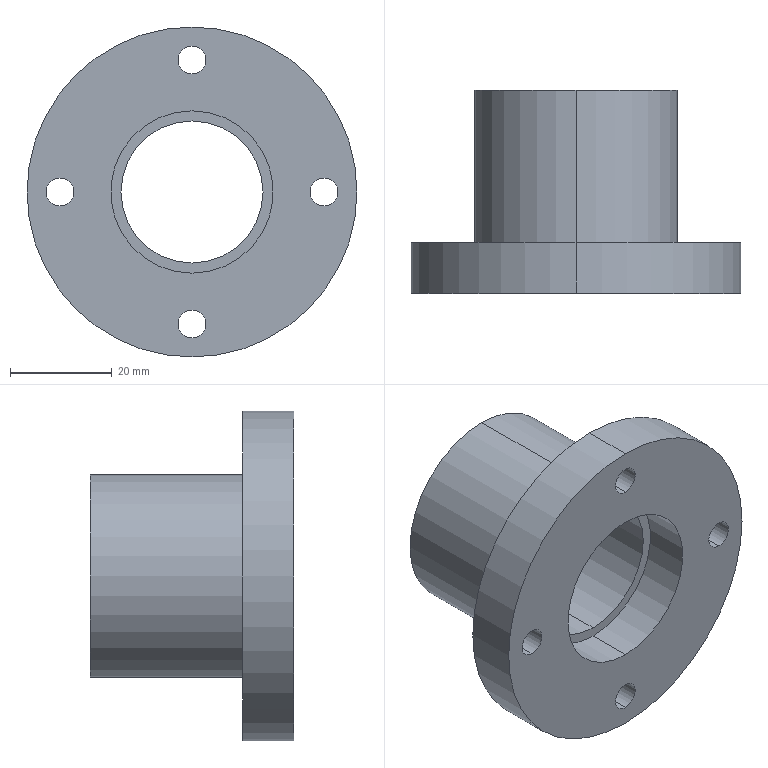Component | SolidWorks | 75-02-23StirringBearingHousing-1 | 1 solid | 35 faces | box 65 x 40 x 65 mm | volume 40660 mm3 | cylinder 26 | plane 9 | commonest cylinder face diameters 10 x8 5.5 x8 32 x4 40 x2 65 x2 28 x2 | material A3 Steel
build123d program:
from build123d import *

# Parameters (mm, degrees)
SKETCH1_R                                          = 32.5
BOSS_EXTRUDE1_DEPTH                                = 10
HOLE_SIZE_ACCORDING_TO_TYPE_OF_HEXAGON_D           = 5.5
HOLE_SIZE_ACCORDING_TO_TYPE_OF_HEXAGON_CBORE_D     = 10
HOLE_SIZE_ACCORDING_TO_TYPE_OF_HEXAGON_CBORE_DEPTH = 5.7
CIRPATTERN1_COUNT                                  = 4
SKETCH5_R                                          = 20
BOSS_EXTRUDE2_DEPTH                                = 30
SKETCH6_R                                          = 14
CUT_EXTRUDE1_DEPTH                                 = 61.93
SKETCH7_R                                          = 16
CUT_EXTRUDE2_DEPTH                                 = 9
CUT_EXTRUDE3_START                                 = -9
SKETCH8_R                                          = 16
CUT_EXTRUDE3_DEPTH                                 = 9


with BuildPart() as part:
    # Sketch1 → Boss-Extrude1 (new body)
    with BuildSketch(Plane.XY):
        Circle(SKETCH1_R)
    extrude(amount=BOSS_EXTRUDE1_DEPTH)

    # Hole Size _according to_ Type of Hexagon (through all)
    with Locations(Plane(origin=(26, 0, 0), x_dir=(-1, 0, 0), z_dir=(0, 0, -1))):
        with Locations((0, 0)):
            hole_size_according_to_type_of_hexagon = CounterBoreHole(HOLE_SIZE_ACCORDING_TO_TYPE_OF_HEXAGON_D / 2, HOLE_SIZE_ACCORDING_TO_TYPE_OF_HEXAGON_CBORE_D / 2, HOLE_SIZE_ACCORDING_TO_TYPE_OF_HEXAGON_CBORE_DEPTH)

    # CirPattern1: Hole Size _according to_ Type of Hexagon ×4 about axis
    cirpattern1_axis = Axis((0, 0, 0), (0, 0, 1))
    for i in range(1, CIRPATTERN1_COUNT):
        add(hole_size_according_to_type_of_hexagon.rotate(cirpattern1_axis, i * 360 / CIRPATTERN1_COUNT), mode=Mode.SUBTRACT)

    # Sketch5 → Boss-Extrude2 (add)
    with BuildSketch(Plane(origin=(0, 0, 0), x_dir=(-1, 0, 0), z_dir=(0, 0, -1))):
        with Locations(Location((0, 0, 0), (0, 0, 180))):
            Circle(SKETCH5_R)
    extrude(amount=BOSS_EXTRUDE2_DEPTH)

    # Sketch6 → Cut-Extrude1 (cut, through all)
    with BuildSketch(Plane(origin=(0, 0, -30), x_dir=(-1, 0, 0), z_dir=(0, 0, -1))):
        Circle(SKETCH6_R)
    extrude(amount=-CUT_EXTRUDE1_DEPTH, mode=Mode.SUBTRACT)

    # Sketch7 → Cut-Extrude2 (cut)
    with BuildSketch(Plane(origin=(0, 0, -30), x_dir=(-1, 0, 0), z_dir=(0, 0, -1))):
        Circle(SKETCH7_R)
    extrude(amount=-CUT_EXTRUDE2_DEPTH, mode=Mode.SUBTRACT)

    # Sketch8 → Cut-Extrude3 (cut)
    with BuildSketch(Plane.XY.offset(10).offset(CUT_EXTRUDE3_START)):
        with Locations(Location((0, 0, 0), (0, 0, 180))):
            Circle(SKETCH8_R)
    extrude(amount=CUT_EXTRUDE3_DEPTH, mode=Mode.SUBTRACT)


solid = part.part

# Placed as in the assembly
solid = solid.moved(Location((-17.87, 205.857, -43.68), (90, 0, 0)))
STEP:
#1=CARTESIAN_POINT('',(-0.7036,8.065,-2.35));
#2=VERTEX_POINT('',#1);
#3=CARTESIAN_POINT('',(-0.7036,8.065,-1.09));
#4=VERTEX_POINT('',#3);
#5=CARTESIAN_POINT('',(-0.7036,8.065,-1.72));
#6=DIRECTION('',(-0.,-1.,0.));
#7=DIRECTION('',(0.,0.,1.));
#8=AXIS2_PLACEMENT_3D('',#5,#6,#7);
#9=CIRCLE('',#8,0.6299);
#10=EDGE_CURVE('',#2,#4,#9,.T.);
#11=ORIENTED_EDGE('',*,*,#10,.F.);
#12=CARTESIAN_POINT('',(-0.7036,7.711,-2.35));
#13=VERTEX_POINT('',#12);
#14=CARTESIAN_POINT('',(-0.7036,8.065,-2.35));
#15=DIRECTION('',(-0.,-1.,0.));
#16=VECTOR('',#15,39.37);
#17=LINE('',#14,#16);
#18=EDGE_CURVE('',#2,#13,#17,.T.);
#19=ORIENTED_EDGE('',*,*,#18,.T.);
#20=CARTESIAN_POINT('',(-0.7036,7.711,-1.09));
#21=VERTEX_POINT('',#20);
#22=CARTESIAN_POINT('',(-0.7036,7.711,-1.72));
#23=DIRECTION('',(-0.,-1.,0.));
#24=DIRECTION('',(0.,0.,1.));
#25=AXIS2_PLACEMENT_3D('',#22,#23,#24);
#26=CIRCLE('',#25,0.6299);
#27=EDGE_CURVE('',#13,#21,#26,.T.);
#28=ORIENTED_EDGE('',*,*,#27,.T.);
#29=CARTESIAN_POINT('',(-0.7036,8.065,-1.09));
#30=DIRECTION('',(-0.,-1.,0.));
#31=VECTOR('',#30,39.37);
#32=LINE('',#29,#31);
#33=EDGE_CURVE('',#4,#21,#32,.T.);
#34=ORIENTED_EDGE('',*,*,#33,.F.);
#35=EDGE_LOOP('',(#11,#19,#28,#34));
#36=FACE_OUTER_BOUND('',#35,.T.);
#37=CARTESIAN_POINT('',(-0.7036,8.065,-1.72));
#38=DIRECTION('',(-0.,-1.,0.));
#39=DIRECTION('',(0.,0.,1.));
#40=AXIS2_PLACEMENT_3D('',#37,#38,#39);
#41=CYLINDRICAL_SURFACE('',#40,0.6299);
#42=ADVANCED_FACE('',(#36),#41,.F.);
#43=CARTESIAN_POINT('',(-0.7036,8.931,-1.09));
#44=VERTEX_POINT('',#43);
#45=CARTESIAN_POINT('',(-0.7036,8.931,-2.35));
#46=VERTEX_POINT('',#45);
#47=CARTESIAN_POINT('',(-0.7036,8.931,-1.72));
#48=DIRECTION('',(0.,1.,-0.));
#49=DIRECTION('',(-0.,0.,-1.));
#50=AXIS2_PLACEMENT_3D('',#47,#48,#49);
#51=CIRCLE('',#50,0.6299);
#52=EDGE_CURVE('',#44,#46,#51,.T.);
#53=ORIENTED_EDGE('',*,*,#52,.F.);
#54=CARTESIAN_POINT('',(-0.7036,9.286,-1.09));
#55=VERTEX_POINT('',#54);
#56=CARTESIAN_POINT('',(-0.7036,8.931,-1.09));
#57=DIRECTION('',(0.,1.,-0.));
#58=VECTOR('',#57,39.37);
#59=LINE('',#56,#58);
#60=EDGE_CURVE('',#44,#55,#59,.T.);
#61=ORIENTED_EDGE('',*,*,#60,.T.);
#62=CARTESIAN_POINT('',(-0.7036,9.286,-2.35));
#63=VERTEX_POINT('',#62);
#64=CARTESIAN_POINT('',(-0.7036,9.286,-1.72));
#65=DIRECTION('',(0.,1.,-0.));
#66=DIRECTION('',(-0.,0.,-1.));
#67=AXIS2_PLACEMENT_3D('',#64,#65,#66);
#68=CIRCLE('',#67,0.6299);
#69=EDGE_CURVE('',#55,#63,#68,.T.);
#70=ORIENTED_EDGE('',*,*,#69,.T.);
#71=CARTESIAN_POINT('',(-0.7036,8.931,-2.35));
#72=DIRECTION('',(0.,1.,-0.));
#73=VECTOR('',#72,39.37);
#74=LINE('',#71,#73);
#75=EDGE_CURVE('',#46,#63,#74,.T.);
#76=ORIENTED_EDGE('',*,*,#75,.F.);
#77=EDGE_LOOP('',(#53,#61,#70,#76));
#78=FACE_OUTER_BOUND('',#77,.T.);
#79=CARTESIAN_POINT('',(-0.7036,8.931,-1.72));
#80=DIRECTION('',(0.,1.,-0.));
#81=DIRECTION('',(-0.,0.,-1.));
#82=AXIS2_PLACEMENT_3D('',#79,#80,#81);
#83=CYLINDRICAL_SURFACE('',#82,0.6299);
#84=ADVANCED_FACE('',(#78),#83,.F.);
#85=CARTESIAN_POINT('',(-0.7036,9.286,-2.507));
#86=VERTEX_POINT('',#85);
#87=CARTESIAN_POINT('',(-0.7036,9.286,-0.9323));
#88=VERTEX_POINT('',#87);
#89=CARTESIAN_POINT('',(-0.7036,9.286,-1.72));
#90=DIRECTION('',(0.,1.,-0.));
#91=DIRECTION('',(-0.,0.,-1.));
#92=AXIS2_PLACEMENT_3D('',#89,#90,#91);
#93=CIRCLE('',#92,0.7874);
#94=EDGE_CURVE('',#86,#88,#93,.T.);
#95=ORIENTED_EDGE('',*,*,#94,.F.);
#96=CARTESIAN_POINT('',(-0.7036,8.105,-2.507));
#97=VERTEX_POINT('',#96);
#98=CARTESIAN_POINT('',(-0.7036,9.286,-2.507));
#99=DIRECTION('',(-0.,-1.,0.));
#100=VECTOR('',#99,39.37);
#101=LINE('',#98,#100);
#102=EDGE_CURVE('',#86,#97,#101,.T.);
#103=ORIENTED_EDGE('',*,*,#102,.T.);
#104=CARTESIAN_POINT('',(-0.7036,8.105,-0.9323));
#105=VERTEX_POINT('',#104);
#106=CARTESIAN_POINT('',(-0.7036,8.105,-1.72));
#107=DIRECTION('',(0.,1.,-0.));
#108=DIRECTION('',(0.,0.,1.));
#109=AXIS2_PLACEMENT_3D('',#106,#107,#108);
#110=CIRCLE('',#109,0.7874);
#111=EDGE_CURVE('',#97,#105,#110,.T.);
#112=ORIENTED_EDGE('',*,*,#111,.T.);
#113=CARTESIAN_POINT('',(-0.7036,9.286,-0.9323));
#114=DIRECTION('',(-0.,-1.,0.));
#115=VECTOR('',#114,39.37);
#116=LINE('',#113,#115);
#117=EDGE_CURVE('',#88,#105,#116,.T.);
#118=ORIENTED_EDGE('',*,*,#117,.F.);
#119=EDGE_LOOP('',(#95,#103,#112,#118));
#120=FACE_OUTER_BOUND('',#119,.T.);
#121=CARTESIAN_POINT('',(-0.7036,9.286,-1.72));
#122=DIRECTION('',(-0.,-1.,0.));
#123=DIRECTION('',(0.,0.,1.));
#124=AXIS2_PLACEMENT_3D('',#121,#122,#123);
#125=CYLINDRICAL_SURFACE('',#124,0.7874);
#126=ADVANCED_FACE('',(#120),#125,.T.);
#127=CARTESIAN_POINT('',(-1.727,7.88,-1.523));
#128=VERTEX_POINT('',#127);
#129=CARTESIAN_POINT('',(-1.727,7.88,-1.917));
#130=VERTEX_POINT('',#129);
#131=CARTESIAN_POINT('',(-1.727,7.88,-1.72));
#132=DIRECTION('',(0.,1.,-0.));
#133=DIRECTION('',(0.,0.,-1.));
#134=AXIS2_PLACEMENT_3D('',#131,#132,#133);
#135=CIRCLE('',#134,0.1969);
#136=EDGE_CURVE('',#128,#130,#135,.T.);
#137=ORIENTED_EDGE('',*,*,#136,.F.);
#138=CARTESIAN_POINT('',(-1.727,8.105,-1.523));
#139=VERTEX_POINT('',#138);
#140=CARTESIAN_POINT('',(-1.727,8.105,-1.523));
#141=DIRECTION('',(0.,1.,-0.));
#142=VECTOR('',#141,39.37);
#143=LINE('',#140,#142);
#144=EDGE_CURVE('',#128,#139,#143,.T.);
#145=ORIENTED_EDGE('',*,*,#144,.T.);
#146=CARTESIAN_POINT('',(-1.727,8.105,-1.917));
#147=VERTEX_POINT('',#146);
#148=CARTESIAN_POINT('',(-1.727,8.105,-1.72));
#149=DIRECTION('',(0.,1.,-0.));
#150=DIRECTION('',(0.,0.,-1.));
#151=AXIS2_PLACEMENT_3D('',#148,#149,#150);
#152=CIRCLE('',#151,0.1969);
#153=EDGE_CURVE('',#139,#147,#152,.T.);
#154=ORIENTED_EDGE('',*,*,#153,.T.);
#155=CARTESIAN_POINT('',(-1.727,8.105,-1.917));
#156=DIRECTION('',(0.,1.,-0.));
#157=VECTOR('',#156,39.37);
#158=LINE('',#155,#157);
#159=EDGE_CURVE('',#130,#147,#158,.T.);
#160=ORIENTED_EDGE('',*,*,#159,.F.);
#161=EDGE_LOOP('',(#137,#145,#154,#160));
#162=FACE_OUTER_BOUND('',#161,.T.);
#163=CARTESIAN_POINT('',(-1.727,8.105,-1.72));
#164=DIRECTION('',(0.,1.,-0.));
#165=DIRECTION('',(0.,0.,-1.));
#166=AXIS2_PLACEMENT_3D('',#163,#164,#165);
#167=CYLINDRICAL_SURFACE('',#166,0.1969);
#168=ADVANCED_FACE('',(#162),#167,.F.);
#169=CARTESIAN_POINT('',(-1.727,7.711,-1.611));
#170=VERTEX_POINT('',#169);
#171=CARTESIAN_POINT('',(-1.727,7.711,-1.828));
#172=VERTEX_POINT('',#171);
#173=CARTESIAN_POINT('',(-1.727,7.711,-1.72));
#174=DIRECTION('',(0.,1.,-0.));
#175=DIRECTION('',(0.,0.,-1.));
#176=AXIS2_PLACEMENT_3D('',#173,#174,#175);
#177=CIRCLE('',#176,0.1083);
#178=EDGE_CURVE('',#170,#172,#177,.T.);
#179=ORIENTED_EDGE('',*,*,#178,.F.);
#180=CARTESIAN_POINT('',(-1.727,7.88,-1.611));
#181=VERTEX_POINT('',#180);
#182=CARTESIAN_POINT('',(-1.727,8.105,-1.611));
#183=DIRECTION('',(0.,1.,-0.));
#184=VECTOR('',#183,39.37);
#185=LINE('',#182,#184);
#186=EDGE_CURVE('',#170,#181,#185,.T.);
#187=ORIENTED_EDGE('',*,*,#186,.T.);
#188=CARTESIAN_POINT('',(-1.727,7.88,-1.828));
#189=VERTEX_POINT('',#188);
#190=CARTESIAN_POINT('',(-1.727,7.88,-1.72));
#191=DIRECTION('',(0.,1.,-0.));
#192=DIRECTION('',(0.,0.,-1.));
#193=AXIS2_PLACEMENT_3D('',#190,#191,#192);
#194=CIRCLE('',#193,0.1083);
#195=EDGE_CURVE('',#181,#189,#194,.T.);
#196=ORIENTED_EDGE('',*,*,#195,.T.);
#197=CARTESIAN_POINT('',(-1.727,8.105,-1.828));
#198=DIRECTION('',(0.,1.,-0.));
#199=VECTOR('',#198,39.37);
#200=LINE('',#197,#199);
#201=EDGE_CURVE('',#172,#189,#200,.T.);
#202=ORIENTED_EDGE('',*,*,#201,.F.);
#203=EDGE_LOOP('',(#179,#187,#196,#202));
#204=FACE_OUTER_BOUND('',#203,.T.);
#205=CARTESIAN_POINT('',(-1.727,8.105,-1.72));
#206=DIRECTION('',(0.,1.,-0.));
#207=DIRECTION('',(0.,0.,-1.));
#208=AXIS2_PLACEMENT_3D('',#205,#206,#207);
#209=CYLINDRICAL_SURFACE('',#208,0.1083);
#210=ADVANCED_FACE('',(#204),#209,.F.);
#211=CARTESIAN_POINT('',(-0.7036,7.88,-2.546));
#212=VERTEX_POINT('',#211);
#213=CARTESIAN_POINT('',(-0.7036,7.88,-2.94));
#214=VERTEX_POINT('',#213);
#215=CARTESIAN_POINT('',(-0.7036,7.88,-2.743));
#216=DIRECTION('',(0.,1.,-0.));
#217=DIRECTION('',(0.,0.,-1.));
#218=AXIS2_PLACEMENT_3D('',#215,#216,#217);
#219=CIRCLE('',#218,0.1969);
#220=EDGE_CURVE('',#212,#214,#219,.T.);
#221=ORIENTED_EDGE('',*,*,#220,.F.);
#222=CARTESIAN_POINT('',(-0.7036,8.105,-2.546));
#223=VERTEX_POINT('',#222);
#224=CARTESIAN_POINT('',(-0.7036,8.105,-2.546));
#225=DIRECTION('',(0.,1.,-0.));
#226=VECTOR('',#225,39.37);
#227=LINE('',#224,#226);
#228=EDGE_CURVE('',#212,#223,#227,.T.);
#229=ORIENTED_EDGE('',*,*,#228,.T.);
#230=CARTESIAN_POINT('',(-0.7036,8.105,-2.94));
#231=VERTEX_POINT('',#230);
#232=CARTESIAN_POINT('',(-0.7036,8.105,-2.743));
#233=DIRECTION('',(0.,1.,-0.));
#234=DIRECTION('',(0.,0.,-1.));
#235=AXIS2_PLACEMENT_3D('',#232,#233,#234);
#236=CIRCLE('',#235,0.1969);
#237=EDGE_CURVE('',#223,#231,#236,.T.);
#238=ORIENTED_EDGE('',*,*,#237,.T.);
#239=CARTESIAN_POINT('',(-0.7036,8.105,-2.94));
#240=DIRECTION('',(0.,1.,-0.));
#241=VECTOR('',#240,39.37);
#242=LINE('',#239,#241);
#243=EDGE_CURVE('',#214,#231,#242,.T.);
#244=ORIENTED_EDGE('',*,*,#243,.F.);
#245=EDGE_LOOP('',(#221,#229,#238,#244));
#246=FACE_OUTER_BOUND('',#245,.T.);
#247=CARTESIAN_POINT('',(-0.7036,8.105,-2.743));
#248=DIRECTION('',(0.,1.,-0.));
#249=DIRECTION('',(0.,0.,-1.));
#250=AXIS2_PLACEMENT_3D('',#247,#248,#249);
#251=CYLINDRICAL_SURFACE('',#250,0.1969);
#252=ADVANCED_FACE('',(#246),#251,.F.);
#253=CARTESIAN_POINT('',(-0.7036,7.711,-2.635));
#254=VERTEX_POINT('',#253);
#255=CARTESIAN_POINT('',(-0.7036,7.711,-2.852));
#256=VERTEX_POINT('',#255);
#257=CARTESIAN_POINT('',(-0.7036,7.711,-2.743));
#258=DIRECTION('',(0.,1.,-0.));
#259=DIRECTION('',(0.,0.,-1.));
#260=AXIS2_PLACEMENT_3D('',#257,#258,#259);
#261=CIRCLE('',#260,0.1083);
#262=EDGE_CURVE('',#254,#256,#261,.T.);
#263=ORIENTED_EDGE('',*,*,#262,.F.);
#264=CARTESIAN_POINT('',(-0.7036,7.88,-2.635));
#265=VERTEX_POINT('',#264);
#266=CARTESIAN_POINT('',(-0.7036,8.105,-2.635));
#267=DIRECTION('',(0.,1.,-0.));
#268=VECTOR('',#267,39.37);
#269=LINE('',#266,#268);
#270=EDGE_CURVE('',#254,#265,#269,.T.);
#271=ORIENTED_EDGE('',*,*,#270,.T.);
#272=CARTESIAN_POINT('',(-0.7036,7.88,-2.852));
#273=VERTEX_POINT('',#272);
#274=CARTESIAN_POINT('',(-0.7036,7.88,-2.743));
#275=DIRECTION('',(0.,1.,-0.));
#276=DIRECTION('',(0.,0.,-1.));
#277=AXIS2_PLACEMENT_3D('',#274,#275,#276);
#278=CIRCLE('',#277,0.1083);
#279=EDGE_CURVE('',#265,#273,#278,.T.);
#280=ORIENTED_EDGE('',*,*,#279,.T.);
#281=CARTESIAN_POINT('',(-0.7036,8.105,-2.852));
#282=DIRECTION('',(0.,1.,-0.));
#283=VECTOR('',#282,39.37);
#284=LINE('',#281,#283);
#285=EDGE_CURVE('',#256,#273,#284,.T.);
#286=ORIENTED_EDGE('',*,*,#285,.F.);
#287=EDGE_LOOP('',(#263,#271,#280,#286));
#288=FACE_OUTER_BOUND('',#287,.T.);
#289=CARTESIAN_POINT('',(-0.7036,8.105,-2.743));
#290=DIRECTION('',(0.,1.,-0.));
#291=DIRECTION('',(0.,0.,-1.));
#292=AXIS2_PLACEMENT_3D('',#289,#290,#291);
#293=CYLINDRICAL_SURFACE('',#292,0.1083);
#294=ADVANCED_FACE('',(#288),#293,.F.);
#295=CARTESIAN_POINT('',(0.3201,7.88,-1.523));
#296=VERTEX_POINT('',#295);
#297=CARTESIAN_POINT('',(0.3201,7.88,-1.917));
#298=VERTEX_POINT('',#297);
#299=CARTESIAN_POINT('',(0.3201,7.88,-1.72));
#300=DIRECTION('',(0.,1.,-0.));
#301=DIRECTION('',(-0.,0.,-1.));
#302=AXIS2_PLACEMENT_3D('',#299,#300,#301);
#303=CIRCLE('',#302,0.1969);
#304=EDGE_CURVE('',#296,#298,#303,.T.);
#305=ORIENTED_EDGE('',*,*,#304,.F.);
#306=CARTESIAN_POINT('',(0.3201,8.105,-1.523));
#307=VERTEX_POINT('',#306);
#308=CARTESIAN_POINT('',(0.3201,8.105,-1.523));
#309=DIRECTION('',(0.,1.,-0.));
#310=VECTOR('',#309,39.37);
#311=LINE('',#308,#310);
#312=EDGE_CURVE('',#296,#307,#311,.T.);
#313=ORIENTED_EDGE('',*,*,#312,.T.);
#314=CARTESIAN_POINT('',(0.3201,8.105,-1.917));
#315=VERTEX_POINT('',#314);
#316=CARTESIAN_POINT('',(0.3201,8.105,-1.72));
#317=DIRECTION('',(0.,1.,-0.));
#318=DIRECTION('',(-0.,0.,-1.));
#319=AXIS2_PLACEMENT_3D('',#316,#317,#318);
#320=CIRCLE('',#319,0.1969);
#321=EDGE_CURVE('',#307,#315,#320,.T.);
#322=ORIENTED_EDGE('',*,*,#321,.T.);
#323=CARTESIAN_POINT('',(0.3201,8.105,-1.917));
#324=DIRECTION('',(0.,1.,-0.));
#325=VECTOR('',#324,39.37);
#326=LINE('',#323,#325);
#327=EDGE_CURVE('',#298,#315,#326,.T.);
#328=ORIENTED_EDGE('',*,*,#327,.F.);
#329=EDGE_LOOP('',(#305,#313,#322,#328));
#330=FACE_OUTER_BOUND('',#329,.T.);
#331=CARTESIAN_POINT('',(0.3201,8.105,-1.72));
#332=DIRECTION('',(0.,1.,-0.));
#333=DIRECTION('',(-0.,0.,-1.));
#334=AXIS2_PLACEMENT_3D('',#331,#332,#333);
#335=CYLINDRICAL_SURFACE('',#334,0.1969);
#336=ADVANCED_FACE('',(#330),#335,.F.);
#337=CARTESIAN_POINT('',(0.3201,7.711,-1.611));
#338=VERTEX_POINT('',#337);
#339=CARTESIAN_POINT('',(0.3201,7.711,-1.828));
#340=VERTEX_POINT('',#339);
#341=CARTESIAN_POINT('',(0.3201,7.711,-1.72));
#342=DIRECTION('',(0.,1.,-0.));
#343=DIRECTION('',(0.,0.,-1.));
#344=AXIS2_PLACEMENT_3D('',#341,#342,#343);
#345=CIRCLE('',#344,0.1083);
#346=EDGE_CURVE('',#338,#340,#345,.T.);
#347=ORIENTED_EDGE('',*,*,#346,.F.);
#348=CARTESIAN_POINT('',(0.3201,7.88,-1.611));
#349=VERTEX_POINT('',#348);
#350=CARTESIAN_POINT('',(0.3201,8.105,-1.611));
#351=DIRECTION('',(0.,1.,-0.));
#352=VECTOR('',#351,39.37);
#353=LINE('',#350,#352);
#354=EDGE_CURVE('',#338,#349,#353,.T.);
#355=ORIENTED_EDGE('',*,*,#354,.T.);
#356=CARTESIAN_POINT('',(0.3201,7.88,-1.828));
#357=VERTEX_POINT('',#356);
#358=CARTESIAN_POINT('',(0.3201,7.88,-1.72));
#359=DIRECTION('',(0.,1.,-0.));
#360=DIRECTION('',(0.,0.,-1.));
#361=AXIS2_PLACEMENT_3D('',#358,#359,#360);
#362=CIRCLE('',#361,0.1083);
#363=EDGE_CURVE('',#349,#357,#362,.T.);
#364=ORIENTED_EDGE('',*,*,#363,.T.);
#365=CARTESIAN_POINT('',(0.3201,8.105,-1.828));
#366=DIRECTION('',(0.,1.,-0.));
#367=VECTOR('',#366,39.37);
#368=LINE('',#365,#367);
#369=EDGE_CURVE('',#340,#357,#368,.T.);
#370=ORIENTED_EDGE('',*,*,#369,.F.);
#371=EDGE_LOOP('',(#347,#355,#364,#370));
#372=FACE_OUTER_BOUND('',#371,.T.);
#373=CARTESIAN_POINT('',(0.3201,8.105,-1.72));
#374=DIRECTION('',(0.,1.,-0.));
#375=DIRECTION('',(0.,0.,-1.));
#376=AXIS2_PLACEMENT_3D('',#373,#374,#375);
#377=CYLINDRICAL_SURFACE('',#376,0.1083);
#378=ADVANCED_FACE('',(#372),#377,.F.);
#379=CARTESIAN_POINT('',(-0.7036,7.88,-0.4992));
#380=VERTEX_POINT('',#379);
#381=CARTESIAN_POINT('',(-0.7036,7.88,-0.8929));
#382=VERTEX_POINT('',#381);
#383=CARTESIAN_POINT('',(-0.7036,7.88,-0.6961));
#384=DIRECTION('',(0.,1.,-0.));
#385=DIRECTION('',(0.,0.,-1.));
#386=AXIS2_PLACEMENT_3D('',#383,#384,#385);
#387=CIRCLE('',#386,0.1969);
#388=EDGE_CURVE('',#380,#382,#387,.T.);
#389=ORIENTED_EDGE('',*,*,#388,.F.);
#390=CARTESIAN_POINT('',(-0.7036,8.105,-0.4992));
#391=VERTEX_POINT('',#390);
#392=CARTESIAN_POINT('',(-0.7036,8.105,-0.4992));
#393=DIRECTION('',(0.,1.,-0.));
#394=VECTOR('',#393,39.37);
#395=LINE('',#392,#394);
#396=EDGE_CURVE('',#380,#391,#395,.T.);
#397=ORIENTED_EDGE('',*,*,#396,.T.);
#398=CARTESIAN_POINT('',(-0.7036,8.105,-0.8929));
#399=VERTEX_POINT('',#398);
#400=CARTESIAN_POINT('',(-0.7036,8.105,-0.6961));
#401=DIRECTION('',(0.,1.,-0.));
#402=DIRECTION('',(0.,0.,-1.));
#403=AXIS2_PLACEMENT_3D('',#400,#401,#402);
#404=CIRCLE('',#403,0.1969);
#405=EDGE_CURVE('',#391,#399,#404,.T.);
#406=ORIENTED_EDGE('',*,*,#405,.T.);
#407=CARTESIAN_POINT('',(-0.7036,8.105,-0.8929));
#408=DIRECTION('',(0.,1.,-0.));
#409=VECTOR('',#408,39.37);
#410=LINE('',#407,#409);
#411=EDGE_CURVE('',#382,#399,#410,.T.);
#412=ORIENTED_EDGE('',*,*,#411,.F.);
#413=EDGE_LOOP('',(#389,#397,#406,#412));
#414=FACE_OUTER_BOUND('',#413,.T.);
#415=CARTESIAN_POINT('',(-0.7036,8.105,-0.6961));
#416=DIRECTION('',(0.,1.,-0.));
#417=DIRECTION('',(0.,0.,-1.));
#418=AXIS2_PLACEMENT_3D('',#415,#416,#417);
#419=CYLINDRICAL_SURFACE('',#418,0.1969);
#420=ADVANCED_FACE('',(#414),#419,.F.);
#421=CARTESIAN_POINT('',(-0.7036,7.711,-0.5878));
#422=VERTEX_POINT('',#421);
#423=CARTESIAN_POINT('',(-0.7036,7.711,-0.8043));
#424=VERTEX_POINT('',#423);
#425=CARTESIAN_POINT('',(-0.7036,7.711,-0.6961));
#426=DIRECTION('',(0.,1.,-0.));
#427=DIRECTION('',(0.,0.,-1.));
#428=AXIS2_PLACEMENT_3D('',#425,#426,#427);
#429=CIRCLE('',#428,0.1083);
#430=EDGE_CURVE('',#422,#424,#429,.T.);
#431=ORIENTED_EDGE('',*,*,#430,.F.);
#432=CARTESIAN_POINT('',(-0.7036,7.88,-0.5878));
#433=VERTEX_POINT('',#432);
#434=CARTESIAN_POINT('',(-0.7036,8.105,-0.5878));
#435=DIRECTION('',(0.,1.,-0.));
#436=VECTOR('',#435,39.37);
#437=LINE('',#434,#436);
#438=EDGE_CURVE('',#422,#433,#437,.T.);
#439=ORIENTED_EDGE('',*,*,#438,.T.);
#440=CARTESIAN_POINT('',(-0.7036,7.88,-0.8043));
#441=VERTEX_POINT('',#440);
#442=CARTESIAN_POINT('',(-0.7036,7.88,-0.6961));
#443=DIRECTION('',(0.,1.,-0.));
#444=DIRECTION('',(0.,0.,-1.));
#445=AXIS2_PLACEMENT_3D('',#442,#443,#444);
#446=CIRCLE('',#445,0.1083);
#447=EDGE_CURVE('',#433,#441,#446,.T.);
#448=ORIENTED_EDGE('',*,*,#447,.T.);
#449=CARTESIAN_POINT('',(-0.7036,8.105,-0.8043));
#450=DIRECTION('',(0.,1.,-0.));
#451=VECTOR('',#450,39.37);
#452=LINE('',#449,#451);
#453=EDGE_CURVE('',#424,#441,#452,.T.);
#454=ORIENTED_EDGE('',*,*,#453,.F.);
#455=EDGE_LOOP('',(#431,#439,#448,#454));
#456=FACE_OUTER_BOUND('',#455,.T.);
#457=CARTESIAN_POINT('',(-0.7036,8.105,-0.6961));
#458=DIRECTION('',(0.,1.,-0.));
#459=DIRECTION('',(0.,0.,-1.));
#460=AXIS2_PLACEMENT_3D('',#457,#458,#459);
#461=CYLINDRICAL_SURFACE('',#460,0.1083);
#462=ADVANCED_FACE('',(#456),#461,.F.);
#463=CARTESIAN_POINT('',(-0.7036,7.711,-0.4402));
#464=VERTEX_POINT('',#463);
#465=CARTESIAN_POINT('',(-0.7036,7.711,-2.999));
#466=VERTEX_POINT('',#465);
#467=CARTESIAN_POINT('',(-0.7036,7.711,-1.72));
#468=DIRECTION('',(-0.,-1.,0.));
#469=DIRECTION('',(0.,0.,1.));
#470=AXIS2_PLACEMENT_3D('',#467,#468,#469);
#471=CIRCLE('',#470,1.28);
#472=EDGE_CURVE('',#464,#466,#471,.T.);
#473=ORIENTED_EDGE('',*,*,#472,.F.);
#474=CARTESIAN_POINT('',(-0.7036,8.105,-0.4402));
#475=VERTEX_POINT('',#474);
#476=CARTESIAN_POINT('',(-0.7036,7.711,-0.4402));
#477=DIRECTION('',(0.,1.,-0.));
#478=VECTOR('',#477,39.37);
#479=LINE('',#476,#478);
#480=EDGE_CURVE('',#464,#475,#479,.T.);
#481=ORIENTED_EDGE('',*,*,#480,.T.);
#482=CARTESIAN_POINT('',(-0.7036,8.105,-2.999));
#483=VERTEX_POINT('',#482);
#484=CARTESIAN_POINT('',(-0.7036,8.105,-1.72));
#485=DIRECTION('',(-0.,-1.,0.));
#486=DIRECTION('',(0.,0.,1.));
#487=AXIS2_PLACEMENT_3D('',#484,#485,#486);
#488=CIRCLE('',#487,1.28);
#489=EDGE_CURVE('',#475,#483,#488,.T.);
#490=ORIENTED_EDGE('',*,*,#489,.T.);
#491=CARTESIAN_POINT('',(-0.7036,7.711,-2.999));
#492=DIRECTION('',(0.,1.,-0.));
#493=VECTOR('',#492,39.37);
#494=LINE('',#491,#493);
#495=EDGE_CURVE('',#466,#483,#494,.T.);
#496=ORIENTED_EDGE('',*,*,#495,.F.);
#497=EDGE_LOOP('',(#473,#481,#490,#496));
#498=FACE_OUTER_BOUND('',#497,.T.);
#499=CARTESIAN_POINT('',(-0.7036,7.711,-1.72));
#500=DIRECTION('',(0.,1.,-0.));
#501=DIRECTION('',(-0.,0.,-1.));
#502=AXIS2_PLACEMENT_3D('',#499,#500,#501);
#503=CYLINDRICAL_SURFACE('',#502,1.28);
#504=ADVANCED_FACE('',(#498),#503,.T.);
#505=CARTESIAN_POINT('',(-0.7036,8.065,-1.169));
#506=VERTEX_POINT('',#505);
#507=CARTESIAN_POINT('',(-0.7036,8.065,-2.271));
#508=VERTEX_POINT('',#507);
#509=CARTESIAN_POINT('',(-0.7036,8.065,-1.72));
#510=DIRECTION('',(0.,1.,-0.));
#511=DIRECTION('',(0.,0.,1.));
#512=AXIS2_PLACEMENT_3D('',#509,#510,#511);
#513=CIRCLE('',#512,0.5512);
#514=EDGE_CURVE('',#506,#508,#513,.T.);
#515=ORIENTED_EDGE('',*,*,#514,.F.);
#516=CARTESIAN_POINT('',(-0.7036,8.931,-1.169));
#517=VERTEX_POINT('',#516);
#518=CARTESIAN_POINT('',(-0.7036,7.711,-1.169));
#519=DIRECTION('',(0.,1.,-0.));
#520=VECTOR('',#519,39.37);
#521=LINE('',#518,#520);
#522=EDGE_CURVE('',#506,#517,#521,.T.);
#523=ORIENTED_EDGE('',*,*,#522,.T.);
#524=CARTESIAN_POINT('',(-0.7036,8.931,-2.271));
#525=VERTEX_POINT('',#524);
#526=CARTESIAN_POINT('',(-0.7036,8.931,-1.72));
#527=DIRECTION('',(-0.,-1.,0.));
#528=DIRECTION('',(-0.,0.,-1.));
#529=AXIS2_PLACEMENT_3D('',#526,#527,#528);
#530=CIRCLE('',#529,0.5512);
#531=EDGE_CURVE('',#525,#517,#530,.T.);
#532=ORIENTED_EDGE('',*,*,#531,.F.);
#533=CARTESIAN_POINT('',(-0.7036,7.711,-2.271));
#534=DIRECTION('',(0.,1.,-0.));
#535=VECTOR('',#534,39.37);
#536=LINE('',#533,#535);
#537=EDGE_CURVE('',#508,#525,#536,.T.);
#538=ORIENTED_EDGE('',*,*,#537,.F.);
#539=EDGE_LOOP('',(#515,#523,#532,#538));
#540=FACE_OUTER_BOUND('',#539,.T.);
#541=CARTESIAN_POINT('',(-0.7036,7.711,-1.72));
#542=DIRECTION('',(0.,1.,-0.));
#543=DIRECTION('',(-0.,0.,-1.));
#544=AXIS2_PLACEMENT_3D('',#541,#542,#543);
#545=CYLINDRICAL_SURFACE('',#544,0.5512);
#546=ADVANCED_FACE('',(#540),#545,.F.);
#547=ORIENTED_EDGE('',*,*,#522,.F.);
#548=CARTESIAN_POINT('',(-0.7036,8.065,-1.72));
#549=DIRECTION('',(0.,1.,-0.));
#550=DIRECTION('',(-0.,0.,1.));
#551=AXIS2_PLACEMENT_3D('',#548,#549,#550);
#552=CIRCLE('',#551,0.5512);
#553=EDGE_CURVE('',#508,#506,#552,.T.);
#554=ORIENTED_EDGE('',*,*,#553,.F.);
#555=ORIENTED_EDGE('',*,*,#537,.T.);
#556=CARTESIAN_POINT('',(-0.7036,8.931,-1.72));
#557=DIRECTION('',(-0.,-1.,0.));
#558=DIRECTION('',(-0.,0.,-1.));
#559=AXIS2_PLACEMENT_3D('',#556,#557,#558);
#560=CIRCLE('',#559,0.5512);
#561=EDGE_CURVE('',#517,#525,#560,.T.);
#562=ORIENTED_EDGE('',*,*,#561,.F.);
#563=EDGE_LOOP('',(#547,#554,#555,#562));
#564=FACE_OUTER_BOUND('',#563,.T.);
#565=CARTESIAN_POINT('',(-0.7036,7.711,-1.72));
#566=DIRECTION('',(0.,1.,-0.));
#567=DIRECTION('',(-0.,0.,-1.));
#568=AXIS2_PLACEMENT_3D('',#565,#566,#567);
#569=CYLINDRICAL_SURFACE('',#568,0.5512);
#570=ADVANCED_FACE('',(#564),#569,.F.);
#571=ORIENTED_EDGE('',*,*,#480,.F.);
#572=CARTESIAN_POINT('',(-0.7036,7.711,-1.72));
#573=DIRECTION('',(-0.,-1.,0.));
#574=DIRECTION('',(0.,0.,1.));
#575=AXIS2_PLACEMENT_3D('',#572,#573,#574);
#576=CIRCLE('',#575,1.28);
#577=EDGE_CURVE('',#466,#464,#576,.T.);
#578=ORIENTED_EDGE('',*,*,#577,.F.);
#579=ORIENTED_EDGE('',*,*,#495,.T.);
#580=CARTESIAN_POINT('',(-0.7036,8.105,-1.72));
#581=DIRECTION('',(-0.,-1.,0.));
#582=DIRECTION('',(0.,0.,1.));
#583=AXIS2_PLACEMENT_3D('',#580,#581,#582);
#584=CIRCLE('',#583,1.28);
#585=EDGE_CURVE('',#483,#475,#584,.T.);
#586=ORIENTED_EDGE('',*,*,#585,.T.);
#587=EDGE_LOOP('',(#571,#578,#579,#586));
#588=FACE_OUTER_BOUND('',#587,.T.);
#589=CARTESIAN_POINT('',(-0.7036,7.711,-1.72));
#590=DIRECTION('',(0.,1.,-0.));
#591=DIRECTION('',(-0.,0.,-1.));
#592=AXIS2_PLACEMENT_3D('',#589,#590,#591);
#593=CYLINDRICAL_SURFACE('',#592,1.28);
#594=ADVANCED_FACE('',(#588),#593,.T.);
#595=CARTESIAN_POINT('',(-0.7036,7.711,-1.72));
#596=DIRECTION('',(-0.,-1.,0.));
#597=DIRECTION('',(0.,0.,1.));
#598=AXIS2_PLACEMENT_3D('',#595,#596,#597);
#599=CIRCLE('',#598,0.6299);
#600=EDGE_CURVE('',#21,#13,#599,.T.);
#601=ORIENTED_EDGE('',*,*,#600,.F.);
#602=ORIENTED_EDGE('',*,*,#27,.F.);
#603=EDGE_LOOP('',(#601,#602));
#604=FACE_BOUND('',#603,.T.);
#605=CARTESIAN_POINT('',(-1.727,7.711,-1.72));
#606=DIRECTION('',(0.,1.,-0.));
#607=DIRECTION('',(0.,0.,-1.));
#608=AXIS2_PLACEMENT_3D('',#605,#606,#607);
#609=CIRCLE('',#608,0.1083);
#610=EDGE_CURVE('',#172,#170,#609,.T.);
#611=ORIENTED_EDGE('',*,*,#610,.T.);
#612=ORIENTED_EDGE('',*,*,#178,.T.);
#613=EDGE_LOOP('',(#611,#612));
#614=FACE_BOUND('',#613,.T.);
#615=CARTESIAN_POINT('',(-0.7036,7.711,-2.743));
#616=DIRECTION('',(0.,1.,-0.));
#617=DIRECTION('',(0.,0.,-1.));
#618=AXIS2_PLACEMENT_3D('',#615,#616,#617);
#619=CIRCLE('',#618,0.1083);
#620=EDGE_CURVE('',#256,#254,#619,.T.);
#621=ORIENTED_EDGE('',*,*,#620,.T.);
#622=ORIENTED_EDGE('',*,*,#262,.T.);
#623=EDGE_LOOP('',(#621,#622));
#624=FACE_BOUND('',#623,.T.);
#625=CARTESIAN_POINT('',(0.3201,7.711,-1.72));
#626=DIRECTION('',(0.,1.,-0.));
#627=DIRECTION('',(0.,0.,-1.));
#628=AXIS2_PLACEMENT_3D('',#625,#626,#627);
#629=CIRCLE('',#628,0.1083);
#630=EDGE_CURVE('',#340,#338,#629,.T.);
#631=ORIENTED_EDGE('',*,*,#630,.T.);
#632=ORIENTED_EDGE('',*,*,#346,.T.);
#633=EDGE_LOOP('',(#631,#632));
#634=FACE_BOUND('',#633,.T.);
#635=CARTESIAN_POINT('',(-0.7036,7.711,-0.6961));
#636=DIRECTION('',(0.,1.,-0.));
#637=DIRECTION('',(0.,0.,-1.));
#638=AXIS2_PLACEMENT_3D('',#635,#636,#637);
#639=CIRCLE('',#638,0.1083);
#640=EDGE_CURVE('',#424,#422,#639,.T.);
#641=ORIENTED_EDGE('',*,*,#640,.T.);
#642=ORIENTED_EDGE('',*,*,#430,.T.);
#643=EDGE_LOOP('',(#641,#642));
#644=FACE_BOUND('',#643,.T.);
#645=ORIENTED_EDGE('',*,*,#577,.T.);
#646=ORIENTED_EDGE('',*,*,#472,.T.);
#647=EDGE_LOOP('',(#645,#646));
#648=FACE_OUTER_BOUND('',#647,.T.);
#649=CARTESIAN_POINT('',(-0.7036,7.711,-1.72));
#650=DIRECTION('',(-0.,-1.,0.));
#651=DIRECTION('',(0.,0.,1.));
#652=AXIS2_PLACEMENT_3D('',#649,#650,#651);
#653=PLANE('',#652);
#654=ADVANCED_FACE('',(#604,#614,#624,#634,#644,#648),#653,.T.);
#655=CARTESIAN_POINT('',(-0.7036,8.105,-1.72));
#656=DIRECTION('',(0.,1.,-0.));
#657=DIRECTION('',(0.,0.,1.));
#658=AXIS2_PLACEMENT_3D('',#655,#656,#657);
#659=CIRCLE('',#658,0.7874);
#660=EDGE_CURVE('',#105,#97,#659,.T.);
#661=ORIENTED_EDGE('',*,*,#660,.F.);
#662=ORIENTED_EDGE('',*,*,#111,.F.);
#663=EDGE_LOOP('',(#661,#662));
#664=FACE_BOUND('',#663,.T.);
#665=CARTESIAN_POINT('',(-1.727,8.105,-1.72));
#666=DIRECTION('',(0.,1.,-0.));
#667=DIRECTION('',(0.,0.,-1.));
#668=AXIS2_PLACEMENT_3D('',#665,#666,#667);
#669=CIRCLE('',#668,0.1969);
#670=EDGE_CURVE('',#147,#139,#669,.T.);
#671=ORIENTED_EDGE('',*,*,#670,.F.);
#672=ORIENTED_EDGE('',*,*,#153,.F.);
#673=EDGE_LOOP('',(#671,#672));
#674=FACE_BOUND('',#673,.T.);
#675=CARTESIAN_POINT('',(-0.7036,8.105,-2.743));
#676=DIRECTION('',(0.,1.,-0.));
#677=DIRECTION('',(0.,0.,-1.));
#678=AXIS2_PLACEMENT_3D('',#675,#676,#677);
#679=CIRCLE('',#678,0.1969);
#680=EDGE_CURVE('',#231,#223,#679,.T.);
#681=ORIENTED_EDGE('',*,*,#680,.F.);
#682=ORIENTED_EDGE('',*,*,#237,.F.);
#683=EDGE_LOOP('',(#681,#682));
#684=FACE_BOUND('',#683,.T.);
#685=CARTESIAN_POINT('',(0.3201,8.105,-1.72));
#686=DIRECTION('',(0.,1.,-0.));
#687=DIRECTION('',(-0.,0.,-1.));
#688=AXIS2_PLACEMENT_3D('',#685,#686,#687);
#689=CIRCLE('',#688,0.1969);
#690=EDGE_CURVE('',#315,#307,#689,.T.);
#691=ORIENTED_EDGE('',*,*,#690,.F.);
#692=ORIENTED_EDGE('',*,*,#321,.F.);
#693=EDGE_LOOP('',(#691,#692));
#694=FACE_BOUND('',#693,.T.);
#695=CARTESIAN_POINT('',(-0.7036,8.105,-0.6961));
#696=DIRECTION('',(0.,1.,-0.));
#697=DIRECTION('',(0.,0.,-1.));
#698=AXIS2_PLACEMENT_3D('',#695,#696,#697);
#699=CIRCLE('',#698,0.1969);
#700=EDGE_CURVE('',#399,#391,#699,.T.);
#701=ORIENTED_EDGE('',*,*,#700,.F.);
#702=ORIENTED_EDGE('',*,*,#405,.F.);
#703=EDGE_LOOP('',(#701,#702));
#704=FACE_BOUND('',#703,.T.);
#705=ORIENTED_EDGE('',*,*,#585,.F.);
#706=ORIENTED_EDGE('',*,*,#489,.F.);
#707=EDGE_LOOP('',(#705,#706));
#708=FACE_OUTER_BOUND('',#707,.T.);
#709=CARTESIAN_POINT('',(-0.7036,8.105,-1.72));
#710=DIRECTION('',(-0.,-1.,0.));
#711=DIRECTION('',(0.,0.,1.));
#712=AXIS2_PLACEMENT_3D('',#709,#710,#711);
#713=PLANE('',#712);
#714=ADVANCED_FACE('',(#664,#674,#684,#694,#704,#708),#713,.F.);
#715=ORIENTED_EDGE('',*,*,#438,.F.);
#716=ORIENTED_EDGE('',*,*,#640,.F.);
#717=ORIENTED_EDGE('',*,*,#453,.T.);
#718=CARTESIAN_POINT('',(-0.7036,7.88,-0.6961));
#719=DIRECTION('',(0.,1.,-0.));
#720=DIRECTION('',(0.,0.,-1.));
#721=AXIS2_PLACEMENT_3D('',#718,#719,#720);
#722=CIRCLE('',#721,0.1083);
#723=EDGE_CURVE('',#441,#433,#722,.T.);
#724=ORIENTED_EDGE('',*,*,#723,.T.);
#725=EDGE_LOOP('',(#715,#716,#717,#724));
#726=FACE_OUTER_BOUND('',#725,.T.);
#727=CARTESIAN_POINT('',(-0.7036,8.105,-0.6961));
#728=DIRECTION('',(0.,1.,-0.));
#729=DIRECTION('',(0.,0.,-1.));
#730=AXIS2_PLACEMENT_3D('',#727,#728,#729);
#731=CYLINDRICAL_SURFACE('',#730,0.1083);
#732=ADVANCED_FACE('',(#726),#731,.F.);
#733=ORIENTED_EDGE('',*,*,#723,.F.);
#734=ORIENTED_EDGE('',*,*,#447,.F.);
#735=EDGE_LOOP('',(#733,#734));
#736=FACE_BOUND('',#735,.T.);
#737=CARTESIAN_POINT('',(-0.7036,7.88,-0.6961));
#738=DIRECTION('',(0.,1.,-0.));
#739=DIRECTION('',(0.,0.,-1.));
#740=AXIS2_PLACEMENT_3D('',#737,#738,#739);
#741=CIRCLE('',#740,0.1969);
#742=EDGE_CURVE('',#382,#380,#741,.T.);
#743=ORIENTED_EDGE('',*,*,#742,.T.);
#744=ORIENTED_EDGE('',*,*,#388,.T.);
#745=EDGE_LOOP('',(#743,#744));
#746=FACE_OUTER_BOUND('',#745,.T.);
#747=CARTESIAN_POINT('',(-0.7036,7.88,-0.5878));
#748=DIRECTION('',(-0.,-1.,0.));
#749=DIRECTION('',(0.,0.,1.));
#750=AXIS2_PLACEMENT_3D('',#747,#748,#749);
#751=PLANE('',#750);
#752=ADVANCED_FACE('',(#736,#746),#751,.F.);
#753=ORIENTED_EDGE('',*,*,#396,.F.);
#754=ORIENTED_EDGE('',*,*,#742,.F.);
#755=ORIENTED_EDGE('',*,*,#411,.T.);
#756=ORIENTED_EDGE('',*,*,#700,.T.);
#757=EDGE_LOOP('',(#753,#754,#755,#756));
#758=FACE_OUTER_BOUND('',#757,.T.);
#759=CARTESIAN_POINT('',(-0.7036,8.105,-0.6961));
#760=DIRECTION('',(0.,1.,-0.));
#761=DIRECTION('',(0.,0.,-1.));
#762=AXIS2_PLACEMENT_3D('',#759,#760,#761);
#763=CYLINDRICAL_SURFACE('',#762,0.1969);
#764=ADVANCED_FACE('',(#758),#763,.F.);
#765=ORIENTED_EDGE('',*,*,#354,.F.);
#766=ORIENTED_EDGE('',*,*,#630,.F.);
#767=ORIENTED_EDGE('',*,*,#369,.T.);
#768=CARTESIAN_POINT('',(0.3201,7.88,-1.72));
#769=DIRECTION('',(0.,1.,-0.));
#770=DIRECTION('',(0.,0.,-1.));
#771=AXIS2_PLACEMENT_3D('',#768,#769,#770);
#772=CIRCLE('',#771,0.1083);
#773=EDGE_CURVE('',#357,#349,#772,.T.);
#774=ORIENTED_EDGE('',*,*,#773,.T.);
#775=EDGE_LOOP('',(#765,#766,#767,#774));
#776=FACE_OUTER_BOUND('',#775,.T.);
#777=CARTESIAN_POINT('',(0.3201,8.105,-1.72));
#778=DIRECTION('',(0.,1.,-0.));
#779=DIRECTION('',(0.,0.,-1.));
#780=AXIS2_PLACEMENT_3D('',#777,#778,#779);
#781=CYLINDRICAL_SURFACE('',#780,0.1083);
#782=ADVANCED_FACE('',(#776),#781,.F.);
#783=ORIENTED_EDGE('',*,*,#773,.F.);
#784=ORIENTED_EDGE('',*,*,#363,.F.);
#785=EDGE_LOOP('',(#783,#784));
#786=FACE_BOUND('',#785,.T.);
#787=CARTESIAN_POINT('',(0.3201,7.88,-1.72));
#788=DIRECTION('',(0.,1.,-0.));
#789=DIRECTION('',(-0.,0.,-1.));
#790=AXIS2_PLACEMENT_3D('',#787,#788,#789);
#791=CIRCLE('',#790,0.1969);
#792=EDGE_CURVE('',#298,#296,#791,.T.);
#793=ORIENTED_EDGE('',*,*,#792,.T.);
#794=ORIENTED_EDGE('',*,*,#304,.T.);
#795=EDGE_LOOP('',(#793,#794));
#796=FACE_OUTER_BOUND('',#795,.T.);
#797=CARTESIAN_POINT('',(0.3201,7.88,-1.611));
#798=DIRECTION('',(-0.,-1.,0.));
#799=DIRECTION('',(0.,0.,1.));
#800=AXIS2_PLACEMENT_3D('',#797,#798,#799);
#801=PLANE('',#800);
#802=ADVANCED_FACE('',(#786,#796),#801,.F.);
#803=ORIENTED_EDGE('',*,*,#312,.F.);
#804=ORIENTED_EDGE('',*,*,#792,.F.);
#805=ORIENTED_EDGE('',*,*,#327,.T.);
#806=ORIENTED_EDGE('',*,*,#690,.T.);
#807=EDGE_LOOP('',(#803,#804,#805,#806));
#808=FACE_OUTER_BOUND('',#807,.T.);
#809=CARTESIAN_POINT('',(0.3201,8.105,-1.72));
#810=DIRECTION('',(0.,1.,-0.));
#811=DIRECTION('',(-0.,0.,-1.));
#812=AXIS2_PLACEMENT_3D('',#809,#810,#811);
#813=CYLINDRICAL_SURFACE('',#812,0.1969);
#814=ADVANCED_FACE('',(#808),#813,.F.);
#815=ORIENTED_EDGE('',*,*,#270,.F.);
#816=ORIENTED_EDGE('',*,*,#620,.F.);
#817=ORIENTED_EDGE('',*,*,#285,.T.);
#818=CARTESIAN_POINT('',(-0.7036,7.88,-2.743));
#819=DIRECTION('',(0.,1.,-0.));
#820=DIRECTION('',(0.,0.,-1.));
#821=AXIS2_PLACEMENT_3D('',#818,#819,#820);
#822=CIRCLE('',#821,0.1083);
#823=EDGE_CURVE('',#273,#265,#822,.T.);
#824=ORIENTED_EDGE('',*,*,#823,.T.);
#825=EDGE_LOOP('',(#815,#816,#817,#824));
#826=FACE_OUTER_BOUND('',#825,.T.);
#827=CARTESIAN_POINT('',(-0.7036,8.105,-2.743));
#828=DIRECTION('',(0.,1.,-0.));
#829=DIRECTION('',(0.,0.,-1.));
#830=AXIS2_PLACEMENT_3D('',#827,#828,#829);
#831=CYLINDRICAL_SURFACE('',#830,0.1083);
#832=ADVANCED_FACE('',(#826),#831,.F.);
#833=ORIENTED_EDGE('',*,*,#823,.F.);
#834=ORIENTED_EDGE('',*,*,#279,.F.);
#835=EDGE_LOOP('',(#833,#834));
#836=FACE_BOUND('',#835,.T.);
#837=CARTESIAN_POINT('',(-0.7036,7.88,-2.743));
#838=DIRECTION('',(0.,1.,-0.));
#839=DIRECTION('',(0.,0.,-1.));
#840=AXIS2_PLACEMENT_3D('',#837,#838,#839);
#841=CIRCLE('',#840,0.1969);
#842=EDGE_CURVE('',#214,#212,#841,.T.);
#843=ORIENTED_EDGE('',*,*,#842,.T.);
#844=ORIENTED_EDGE('',*,*,#220,.T.);
#845=EDGE_LOOP('',(#843,#844));
#846=FACE_OUTER_BOUND('',#845,.T.);
#847=CARTESIAN_POINT('',(-0.7036,7.88,-2.635));
#848=DIRECTION('',(-0.,-1.,0.));
#849=DIRECTION('',(0.,0.,1.));
#850=AXIS2_PLACEMENT_3D('',#847,#848,#849);
#851=PLANE('',#850);
#852=ADVANCED_FACE('',(#836,#846),#851,.F.);
#853=ORIENTED_EDGE('',*,*,#228,.F.);
#854=ORIENTED_EDGE('',*,*,#842,.F.);
#855=ORIENTED_EDGE('',*,*,#243,.T.);
#856=ORIENTED_EDGE('',*,*,#680,.T.);
#857=EDGE_LOOP('',(#853,#854,#855,#856));
#858=FACE_OUTER_BOUND('',#857,.T.);
#859=CARTESIAN_POINT('',(-0.7036,8.105,-2.743));
#860=DIRECTION('',(0.,1.,-0.));
#861=DIRECTION('',(0.,0.,-1.));
#862=AXIS2_PLACEMENT_3D('',#859,#860,#861);
#863=CYLINDRICAL_SURFACE('',#862,0.1969);
#864=ADVANCED_FACE('',(#858),#863,.F.);
#865=ORIENTED_EDGE('',*,*,#186,.F.);
#866=ORIENTED_EDGE('',*,*,#610,.F.);
#867=ORIENTED_EDGE('',*,*,#201,.T.);
#868=CARTESIAN_POINT('',(-1.727,7.88,-1.72));
#869=DIRECTION('',(0.,1.,-0.));
#870=DIRECTION('',(0.,0.,-1.));
#871=AXIS2_PLACEMENT_3D('',#868,#869,#870);
#872=CIRCLE('',#871,0.1083);
#873=EDGE_CURVE('',#189,#181,#872,.T.);
#874=ORIENTED_EDGE('',*,*,#873,.T.);
#875=EDGE_LOOP('',(#865,#866,#867,#874));
#876=FACE_OUTER_BOUND('',#875,.T.);
#877=CARTESIAN_POINT('',(-1.727,8.105,-1.72));
#878=DIRECTION('',(0.,1.,-0.));
#879=DIRECTION('',(0.,0.,-1.));
#880=AXIS2_PLACEMENT_3D('',#877,#878,#879);
#881=CYLINDRICAL_SURFACE('',#880,0.1083);
#882=ADVANCED_FACE('',(#876),#881,.F.);
#883=ORIENTED_EDGE('',*,*,#873,.F.);
#884=ORIENTED_EDGE('',*,*,#195,.F.);
#885=EDGE_LOOP('',(#883,#884));
#886=FACE_BOUND('',#885,.T.);
#887=CARTESIAN_POINT('',(-1.727,7.88,-1.72));
#888=DIRECTION('',(0.,1.,-0.));
#889=DIRECTION('',(0.,0.,-1.));
#890=AXIS2_PLACEMENT_3D('',#887,#888,#889);
#891=CIRCLE('',#890,0.1969);
#892=EDGE_CURVE('',#130,#128,#891,.T.);
#893=ORIENTED_EDGE('',*,*,#892,.T.);
#894=ORIENTED_EDGE('',*,*,#136,.T.);
#895=EDGE_LOOP('',(#893,#894));
#896=FACE_OUTER_BOUND('',#895,.T.);
#897=CARTESIAN_POINT('',(-1.727,7.88,-1.611));
#898=DIRECTION('',(-0.,-1.,0.));
#899=DIRECTION('',(0.,0.,1.));
#900=AXIS2_PLACEMENT_3D('',#897,#898,#899);
#901=PLANE('',#900);
#902=ADVANCED_FACE('',(#886,#896),#901,.F.);
#903=ORIENTED_EDGE('',*,*,#144,.F.);
#904=ORIENTED_EDGE('',*,*,#892,.F.);
#905=ORIENTED_EDGE('',*,*,#159,.T.);
#906=ORIENTED_EDGE('',*,*,#670,.T.);
#907=EDGE_LOOP('',(#903,#904,#905,#906));
#908=FACE_OUTER_BOUND('',#907,.T.);
#909=CARTESIAN_POINT('',(-1.727,8.105,-1.72));
#910=DIRECTION('',(0.,1.,-0.));
#911=DIRECTION('',(0.,0.,-1.));
#912=AXIS2_PLACEMENT_3D('',#909,#910,#911);
#913=CYLINDRICAL_SURFACE('',#912,0.1969);
#914=ADVANCED_FACE('',(#908),#913,.F.);
#915=ORIENTED_EDGE('',*,*,#102,.F.);
#916=CARTESIAN_POINT('',(-0.7036,9.286,-1.72));
#917=DIRECTION('',(0.,1.,-0.));
#918=DIRECTION('',(-0.,0.,-1.));
#919=AXIS2_PLACEMENT_3D('',#916,#917,#918);
#920=CIRCLE('',#919,0.7874);
#921=EDGE_CURVE('',#88,#86,#920,.T.);
#922=ORIENTED_EDGE('',*,*,#921,.F.);
#923=ORIENTED_EDGE('',*,*,#117,.T.);
#924=ORIENTED_EDGE('',*,*,#660,.T.);
#925=EDGE_LOOP('',(#915,#922,#923,#924));
#926=FACE_OUTER_BOUND('',#925,.T.);
#927=CARTESIAN_POINT('',(-0.7036,9.286,-1.72));
#928=DIRECTION('',(-0.,-1.,0.));
#929=DIRECTION('',(0.,0.,1.));
#930=AXIS2_PLACEMENT_3D('',#927,#928,#929);
#931=CYLINDRICAL_SURFACE('',#930,0.7874);
#932=ADVANCED_FACE('',(#926),#931,.T.);
#933=CARTESIAN_POINT('',(-0.7036,9.286,-1.72));
#934=DIRECTION('',(0.,1.,-0.));
#935=DIRECTION('',(-0.,0.,-1.));
#936=AXIS2_PLACEMENT_3D('',#933,#934,#935);
#937=CIRCLE('',#936,0.6299);
#938=EDGE_CURVE('',#63,#55,#937,.T.);
#939=ORIENTED_EDGE('',*,*,#938,.F.);
#940=ORIENTED_EDGE('',*,*,#69,.F.);
#941=EDGE_LOOP('',(#939,#940));
#942=FACE_BOUND('',#941,.T.);
#943=ORIENTED_EDGE('',*,*,#921,.T.);
#944=ORIENTED_EDGE('',*,*,#94,.T.);
#945=EDGE_LOOP('',(#943,#944));
#946=FACE_OUTER_BOUND('',#945,.T.);
#947=CARTESIAN_POINT('',(-0.7036,9.286,-1.72));
#948=DIRECTION('',(0.,1.,-0.));
#949=DIRECTION('',(-0.,-0.,-1.));
#950=AXIS2_PLACEMENT_3D('',#947,#948,#949);
#951=PLANE('',#950);
#952=ADVANCED_FACE('',(#942,#946),#951,.T.);
#953=CARTESIAN_POINT('',(-0.7036,8.931,-1.72));
#954=DIRECTION('',(0.,1.,-0.));
#955=DIRECTION('',(-0.,0.,-1.));
#956=AXIS2_PLACEMENT_3D('',#953,#954,#955);
#957=CIRCLE('',#956,0.6299);
#958=EDGE_CURVE('',#46,#44,#957,.T.);
#959=ORIENTED_EDGE('',*,*,#958,.T.);
#960=ORIENTED_EDGE('',*,*,#52,.T.);
#961=EDGE_LOOP('',(#959,#960));
#962=FACE_OUTER_BOUND('',#961,.T.);
#963=ORIENTED_EDGE('',*,*,#531,.T.);
#964=ORIENTED_EDGE('',*,*,#561,.T.);
#965=EDGE_LOOP('',(#963,#964));
#966=FACE_BOUND('',#965,.T.);
#967=CARTESIAN_POINT('',(-0.7036,8.931,-1.72));
#968=DIRECTION('',(0.,1.,-0.));
#969=DIRECTION('',(-0.,-0.,-1.));
#970=AXIS2_PLACEMENT_3D('',#967,#968,#969);
#971=PLANE('',#970);
#972=ADVANCED_FACE('',(#962,#966),#971,.T.);
#973=ORIENTED_EDGE('',*,*,#60,.F.);
#974=ORIENTED_EDGE('',*,*,#958,.F.);
#975=ORIENTED_EDGE('',*,*,#75,.T.);
#976=ORIENTED_EDGE('',*,*,#938,.T.);
#977=EDGE_LOOP('',(#973,#974,#975,#976));
#978=FACE_OUTER_BOUND('',#977,.T.);
#979=CARTESIAN_POINT('',(-0.7036,8.931,-1.72));
#980=DIRECTION('',(0.,1.,-0.));
#981=DIRECTION('',(-0.,0.,-1.));
#982=AXIS2_PLACEMENT_3D('',#979,#980,#981);
#983=CYLINDRICAL_SURFACE('',#982,0.6299);
#984=ADVANCED_FACE('',(#978),#983,.F.);
#985=CARTESIAN_POINT('',(-0.7036,8.065,-1.72));
#986=DIRECTION('',(-0.,-1.,0.));
#987=DIRECTION('',(0.,0.,1.));
#988=AXIS2_PLACEMENT_3D('',#985,#986,#987);
#989=CIRCLE('',#988,0.6299);
#990=EDGE_CURVE('',#4,#2,#989,.T.);
#991=ORIENTED_EDGE('',*,*,#990,.T.);
#992=ORIENTED_EDGE('',*,*,#10,.T.);
#993=EDGE_LOOP('',(#991,#992));
#994=FACE_OUTER_BOUND('',#993,.T.);
#995=ORIENTED_EDGE('',*,*,#553,.T.);
#996=ORIENTED_EDGE('',*,*,#514,.T.);
#997=EDGE_LOOP('',(#995,#996));
#998=FACE_BOUND('',#997,.T.);
#999=CARTESIAN_POINT('',(-0.7036,8.065,-1.72));
#1000=DIRECTION('',(-0.,-1.,0.));
#1001=DIRECTION('',(0.,0.,1.));
#1002=AXIS2_PLACEMENT_3D('',#999,#1000,#1001);
#1003=PLANE('',#1002);
#1004=ADVANCED_FACE('',(#994,#998),#1003,.T.);
#1005=ORIENTED_EDGE('',*,*,#18,.F.);
#1006=ORIENTED_EDGE('',*,*,#990,.F.);
#1007=ORIENTED_EDGE('',*,*,#33,.T.);
#1008=ORIENTED_EDGE('',*,*,#600,.T.);
#1009=EDGE_LOOP('',(#1005,#1006,#1007,#1008));
#1010=FACE_OUTER_BOUND('',#1009,.T.);
#1011=CARTESIAN_POINT('',(-0.7036,8.065,-1.72));
#1012=DIRECTION('',(-0.,-1.,0.));
#1013=DIRECTION('',(0.,0.,1.));
#1014=AXIS2_PLACEMENT_3D('',#1011,#1012,#1013);
#1015=CYLINDRICAL_SURFACE('',#1014,0.6299);
#1016=ADVANCED_FACE('',(#1010),#1015,.F.);
#1017=CLOSED_SHELL('',(#42,#84,#126,#168,#210,#252,#294,#336,#378,#420,#462,#504,#546,#570,#594,#654,#714,#732,#752,#764,#782,#802,#814,#832,#852,#864,#882,#902,#914,#932,#952,#972,#984,#1004,#1016));
#1018=MANIFOLD_SOLID_BREP('',#1017);
#1019=CARTESIAN_POINT('',(0.,0.,0.));
#1020=DIRECTION('',(0.,0.,1.));
#1021=DIRECTION('',(1.,0.,0.));
#1022=AXIS2_PLACEMENT_3D('',#1019,#1020,#1021);
#1023=(LENGTH_UNIT()NAMED_UNIT(*)SI_UNIT($,.METRE.));
#1024=LENGTH_MEASURE_WITH_UNIT(LENGTH_MEASURE(0.0254),#1023);
#1025=DIMENSIONAL_EXPONENTS(1.,0.,0.,0.,0.,0.,0.);
#1026=(CONVERSION_BASED_UNIT('',#1024)LENGTH_UNIT()NAMED_UNIT(#1025));
#1027=UNCERTAINTY_MEASURE_WITH_UNIT(LENGTH_MEASURE(0.00001),#1026,'','');
#1028=(NAMED_UNIT(*)PLANE_ANGLE_UNIT()SI_UNIT($,.RADIAN.));
#1029=(NAMED_UNIT(*)SI_UNIT($,.STERADIAN.)SOLID_ANGLE_UNIT());
#1030=(GEOMETRIC_REPRESENTATION_CONTEXT(3)GLOBAL_UNCERTAINTY_ASSIGNED_CONTEXT((#1027))GLOBAL_UNIT_ASSIGNED_CONTEXT((#1026,#1028,#1029))REPRESENTATION_CONTEXT('',''));
#1031=ADVANCED_BREP_SHAPE_REPRESENTATION('',(#1018,#1022),#1030);
#1032=COLOUR_RGB('',0.7922,0.8196,0.9333);
#1033=FILL_AREA_STYLE_COLOUR('',#1032);
#1034=FILL_AREA_STYLE('',(#1033));
#1035=SURFACE_STYLE_FILL_AREA(#1034);
#1036=SURFACE_SIDE_STYLE('',(#1035));
#1037=SURFACE_STYLE_USAGE(.BOTH.,#1036);
#1038=PRESENTATION_STYLE_ASSIGNMENT((#1037));
#1039=STYLED_ITEM('',(#1038),#1018);
#1040=(LENGTH_UNIT()NAMED_UNIT(*)SI_UNIT($,.METRE.));
#1041=LENGTH_MEASURE_WITH_UNIT(LENGTH_MEASURE(0.0254),#1040);
#1042=DIMENSIONAL_EXPONENTS(1.,0.,0.,0.,0.,0.,0.);
#1043=(CONVERSION_BASED_UNIT('',#1041)LENGTH_UNIT()NAMED_UNIT(#1042));
#1044=UNCERTAINTY_MEASURE_WITH_UNIT(LENGTH_MEASURE(0.00001),#1043,'','');
#1045=(NAMED_UNIT(*)PLANE_ANGLE_UNIT()SI_UNIT($,.RADIAN.));
#1046=(NAMED_UNIT(*)SI_UNIT($,.STERADIAN.)SOLID_ANGLE_UNIT());
#1047=(GEOMETRIC_REPRESENTATION_CONTEXT(3)GLOBAL_UNCERTAINTY_ASSIGNED_CONTEXT((#1044))GLOBAL_UNIT_ASSIGNED_CONTEXT((#1043,#1045,#1046))REPRESENTATION_CONTEXT('',''));
#1048=MECHANICAL_DESIGN_GEOMETRIC_PRESENTATION_REPRESENTATION('',(#1039),#1047);
#1049=PRESENTATION_LAYER_ASSIGNMENT('','',(#1039));